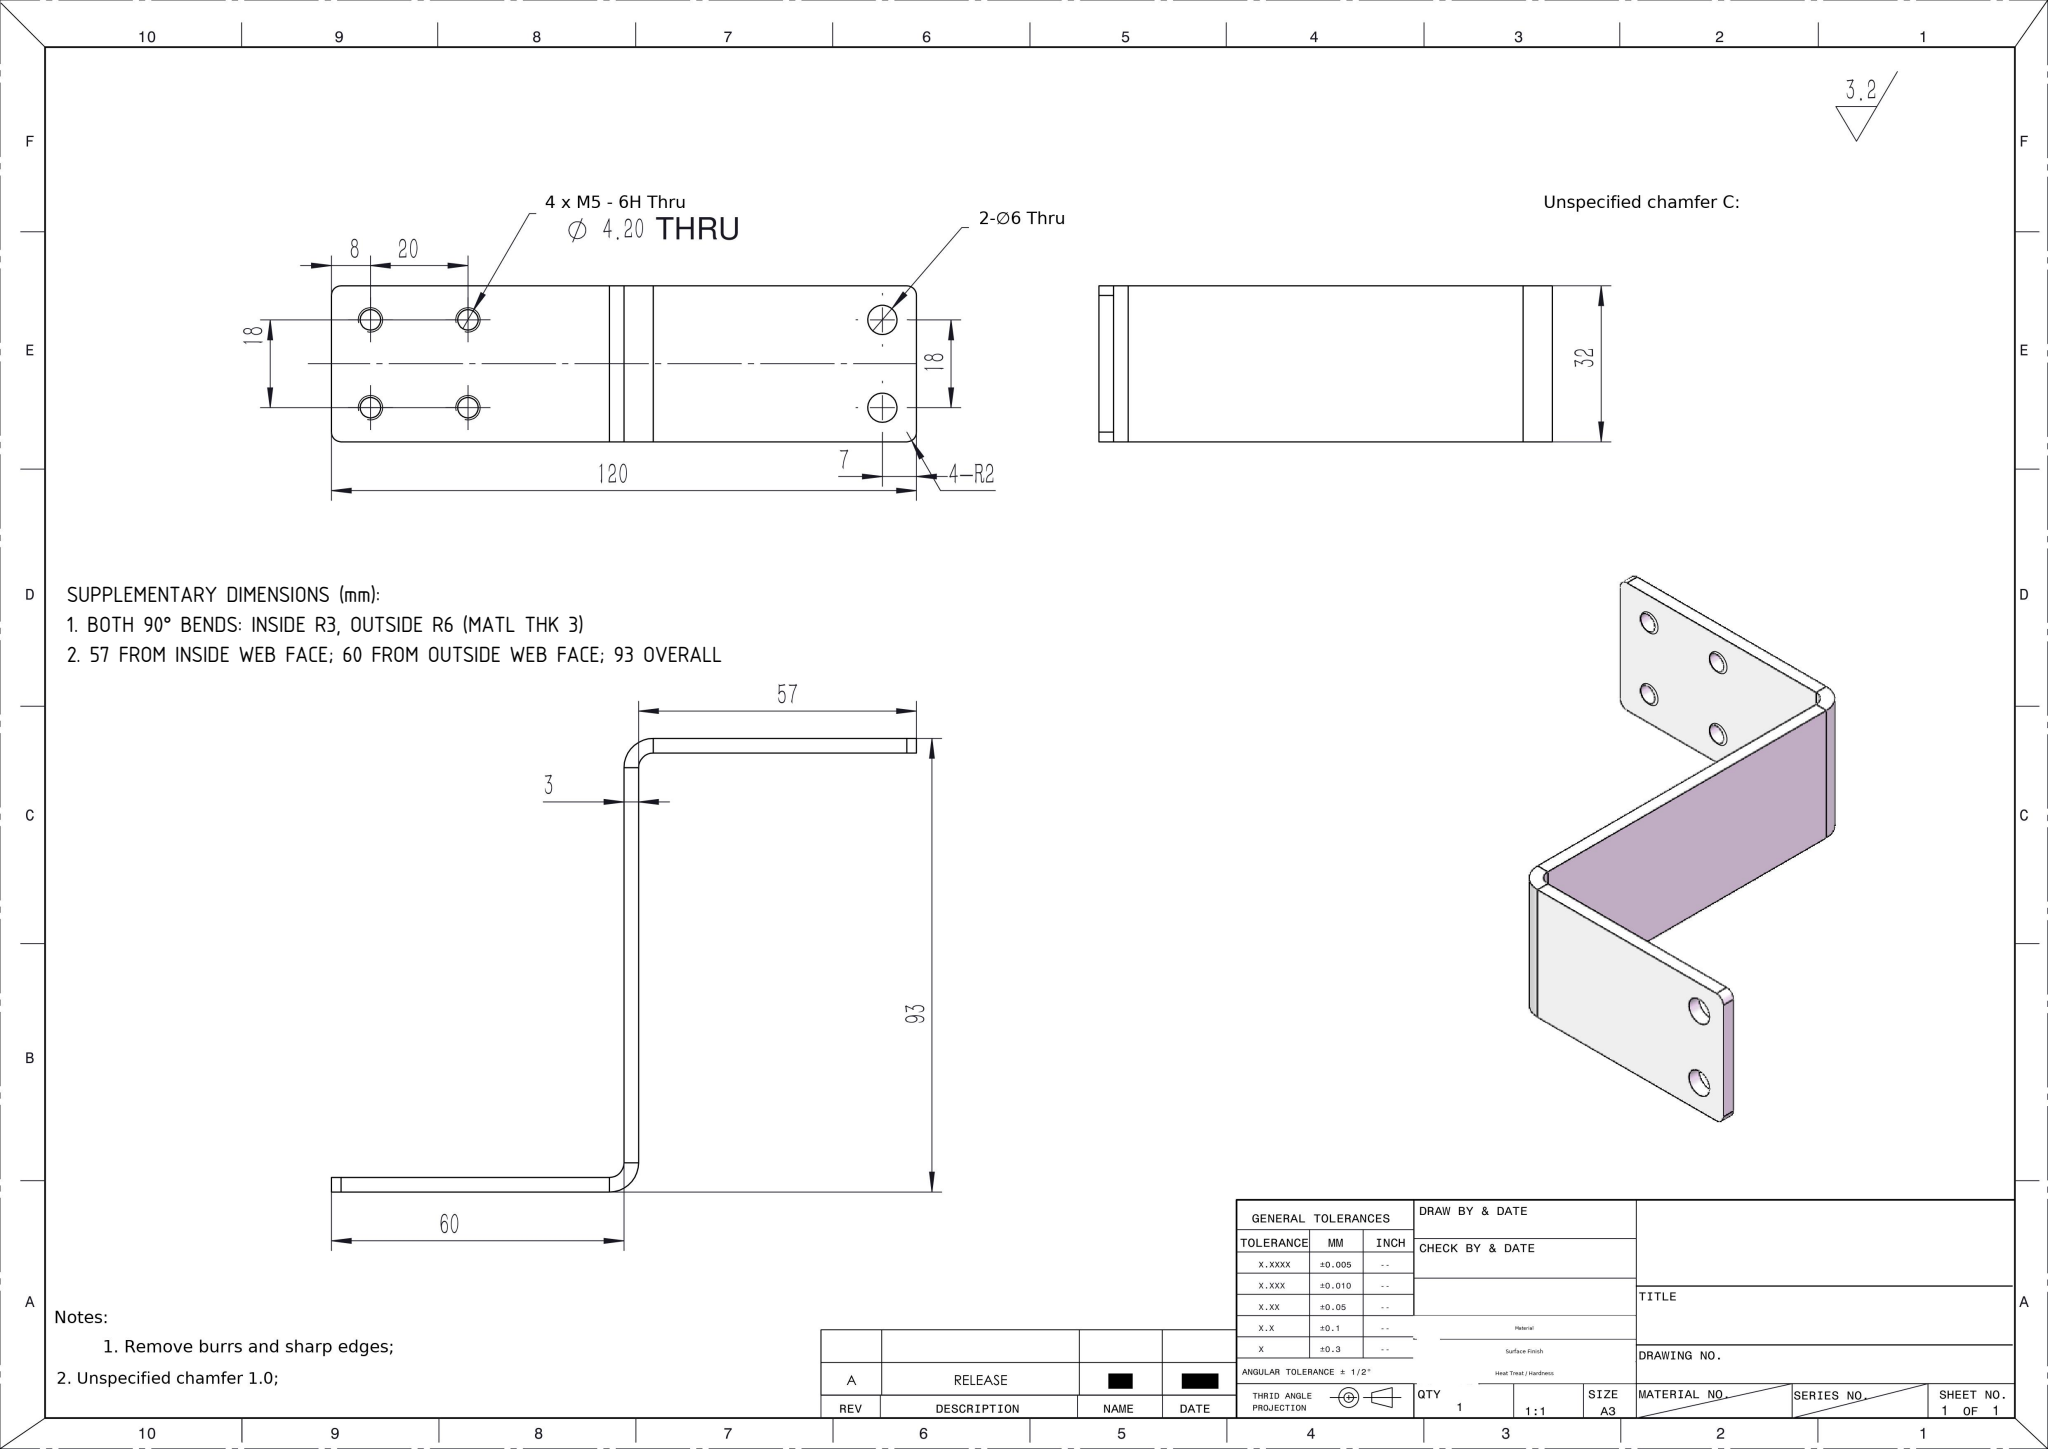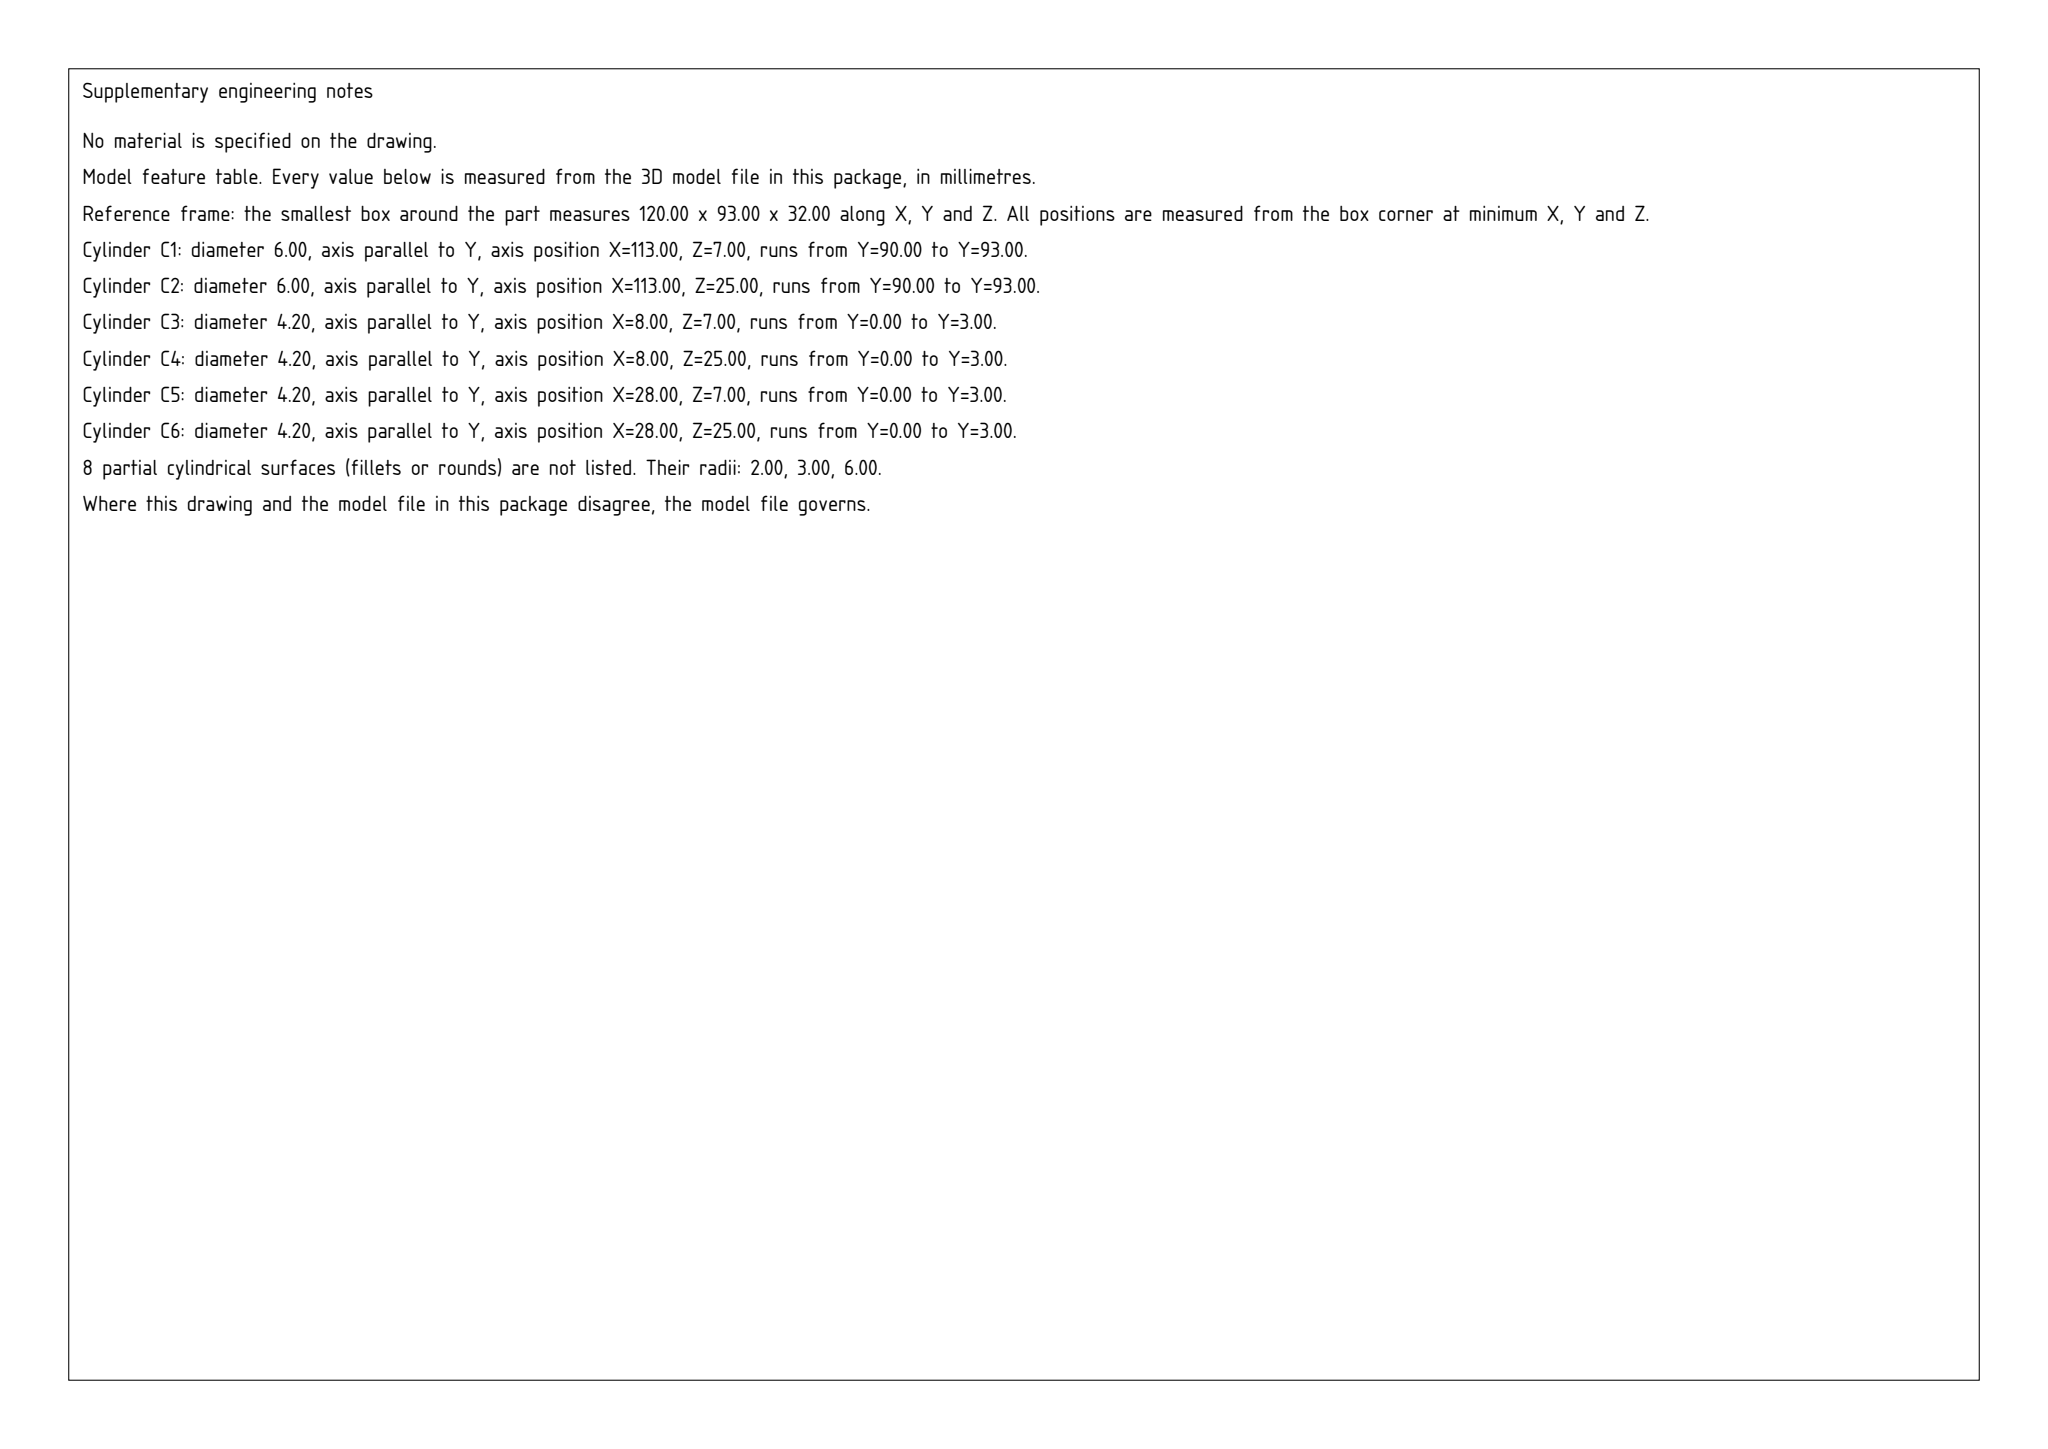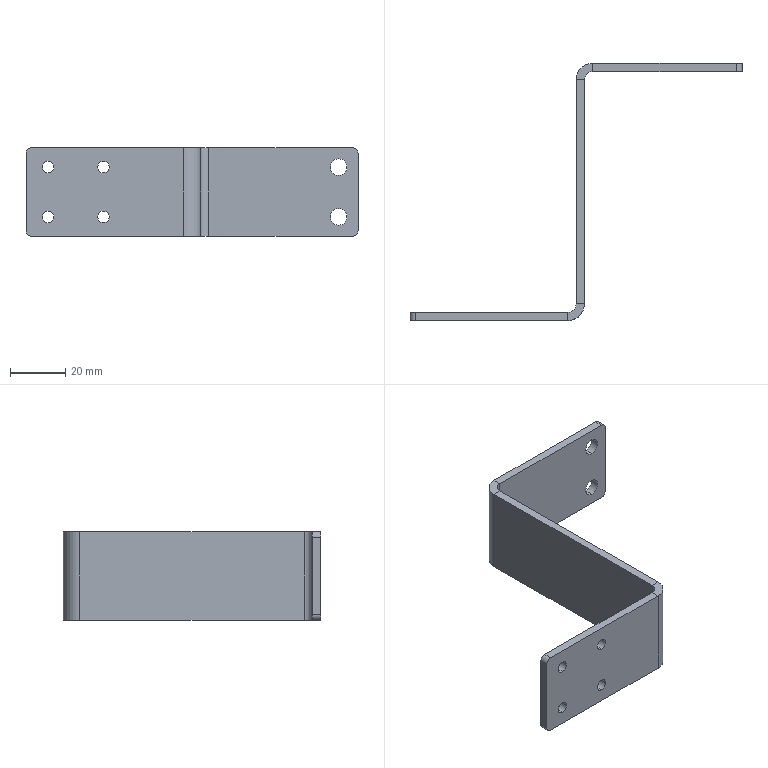Part | SolidWorks | mm | 1 solid | 38 faces | box 120 x 93 x 32 mm | volume 19443 mm3 | cylinder 20 | plane 18 | commonest cylinder face diameters 4.2 x8 6 x6 4 x4 12 x2